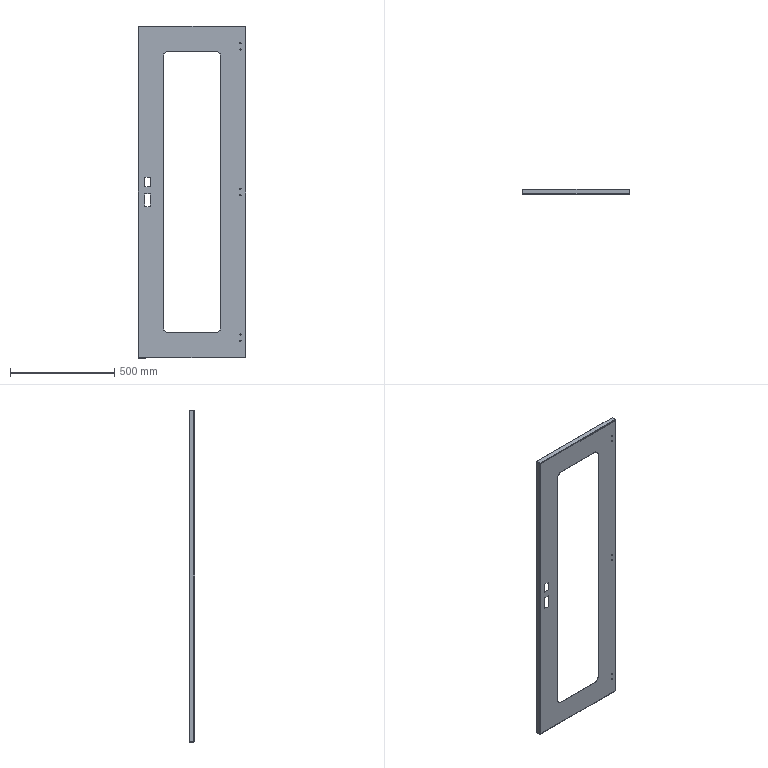Component | SolidWorks | GlassDoorAssembly-1_GlassDoor-1 | 1 solid | 98 faces | volume 1077008 mm3 | plane 74 | cylinder 24 | commonest cylinder face diameters 6 x16 2 x4 50 x4